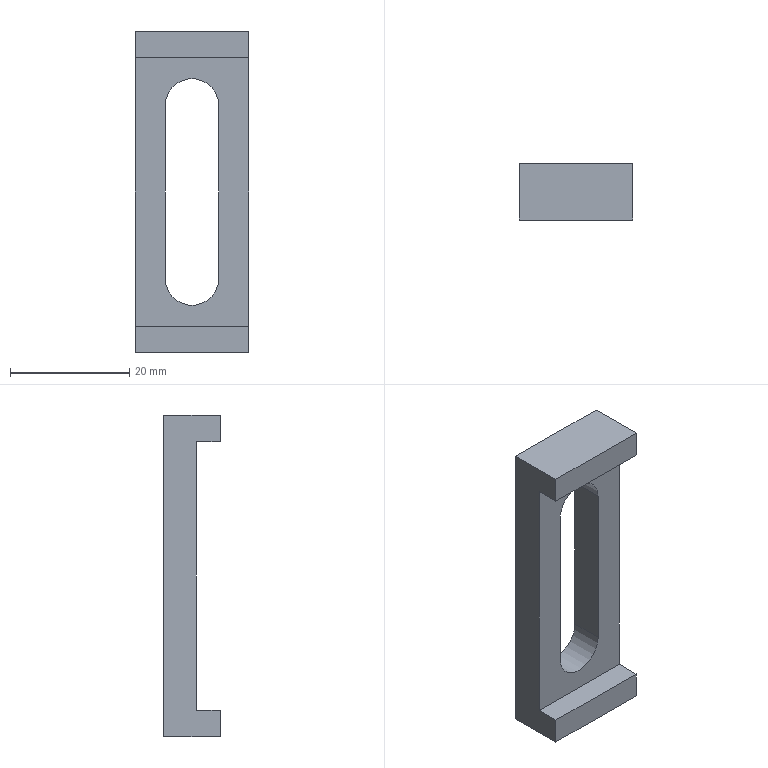Component | NX | SIDE_SUPPORT_FRAME | 1 solid | 14 faces | box 19 x 9.5 x 54 mm | volume 4542 mm3 | plane 12 | cylinder 2 | commonest cylinder face diameters 9 x2
STEP:
#1=CARTESIAN_POINT('',(0.,0.,0.));
#2=DIRECTION('',(0.,0.,1.));
#3=DIRECTION('',(1.,0.,0.));
#4=AXIS2_PLACEMENT_3D('',#1,#2,#3);
#5=CARTESIAN_POINT('',(-95.,46.,111.498));
#6=VERTEX_POINT('',#5);
#7=CARTESIAN_POINT('',(-95.,46.,115.998));
#8=VERTEX_POINT('',#7);
#9=CARTESIAN_POINT('',(-95.,46.,111.498));
#10=DIRECTION('',(0.,0.,1.));
#11=VECTOR('',#10,1.);
#12=LINE('',#9,#11);
#13=CARTESIAN_POINT('',(-104.5,46.,138.498));
#14=DIRECTION('',(0.,-1.,0.));
#15=DIRECTION('',(0.,0.,-1.));
#16=AXIS2_PLACEMENT_3D('',#13,#14,#15);
#17=PLANE('',#16);
#18=CARTESIAN_POINT('',(27.,9.5));
#19=DIRECTION('',(-1.,0.));
#20=VECTOR('',#19,1.);
#21=LINE('',#18,#20);
#22=(GEOMETRIC_REPRESENTATION_CONTEXT(2)PARAMETRIC_REPRESENTATION_CONTEXT()REPRESENTATION_CONTEXT('',''));
#23=DEFINITIONAL_REPRESENTATION('',(#21),#22);
#24=PCURVE('',#17,#23);
#25=CARTESIAN_POINT('',(-95.,46.,111.498));
#26=DIRECTION('',(-1.,0.,0.));
#27=DIRECTION('',(0.,0.,-1.));
#28=AXIS2_PLACEMENT_3D('',#25,#26,#27);
#29=PLANE('',#28);
#30=CARTESIAN_POINT('',(0.,0.));
#31=DIRECTION('',(-1.,0.));
#32=VECTOR('',#31,1.);
#33=LINE('',#30,#32);
#34=(GEOMETRIC_REPRESENTATION_CONTEXT(2)PARAMETRIC_REPRESENTATION_CONTEXT()REPRESENTATION_CONTEXT('',''));
#35=DEFINITIONAL_REPRESENTATION('',(#33),#34);
#36=PCURVE('',#29,#35);
#37=SURFACE_CURVE('',#12,(#24,#36),.PCURVE_S1.);
#38=EDGE_CURVE('',#6,#8,#37,.T.);
#39=ORIENTED_EDGE('',*,*,#38,.T.);
#40=CARTESIAN_POINT('',(-114.,46.,115.998));
#41=VERTEX_POINT('',#40);
#42=CARTESIAN_POINT('',(-94.,46.,115.998));
#43=DIRECTION('',(-1.,0.,0.));
#44=VECTOR('',#43,1.);
#45=LINE('',#42,#44);
#46=CARTESIAN_POINT('',(22.5,10.5));
#47=DIRECTION('',(0.,-1.));
#48=VECTOR('',#47,1.);
#49=LINE('',#46,#48);
#50=(GEOMETRIC_REPRESENTATION_CONTEXT(2)PARAMETRIC_REPRESENTATION_CONTEXT()REPRESENTATION_CONTEXT('',''));
#51=DEFINITIONAL_REPRESENTATION('',(#49),#50);
#52=PCURVE('',#17,#51);
#53=CARTESIAN_POINT('',(-94.,50.,115.998));
#54=DIRECTION('',(0.,0.,-1.));
#55=DIRECTION('',(0.,1.,0.));
#56=AXIS2_PLACEMENT_3D('',#53,#54,#55);
#57=PLANE('',#56);
#58=CARTESIAN_POINT('',(-4.,0.));
#59=DIRECTION('',(0.,-1.));
#60=VECTOR('',#59,1.);
#61=LINE('',#58,#60);
#62=(GEOMETRIC_REPRESENTATION_CONTEXT(2)PARAMETRIC_REPRESENTATION_CONTEXT()REPRESENTATION_CONTEXT('',''));
#63=DEFINITIONAL_REPRESENTATION('',(#61),#62);
#64=PCURVE('',#57,#63);
#65=SURFACE_CURVE('',#45,(#52,#64),.PCURVE_S1.);
#66=EDGE_CURVE('',#8,#41,#65,.T.);
#67=ORIENTED_EDGE('',*,*,#66,.T.);
#68=CARTESIAN_POINT('',(-114.,46.,111.498));
#69=VERTEX_POINT('',#68);
#70=CARTESIAN_POINT('',(-114.,46.,165.498));
#71=DIRECTION('',(0.,0.,-1.));
#72=VECTOR('',#71,1.);
#73=LINE('',#70,#72);
#74=CARTESIAN_POINT('',(-27.,-9.5));
#75=DIRECTION('',(1.,0.));
#76=VECTOR('',#75,1.);
#77=LINE('',#74,#76);
#78=(GEOMETRIC_REPRESENTATION_CONTEXT(2)PARAMETRIC_REPRESENTATION_CONTEXT()REPRESENTATION_CONTEXT('',''));
#79=DEFINITIONAL_REPRESENTATION('',(#77),#78);
#80=PCURVE('',#17,#79);
#81=CARTESIAN_POINT('',(-114.,46.,165.498));
#82=DIRECTION('',(1.,0.,0.));
#83=DIRECTION('',(0.,0.,1.));
#84=AXIS2_PLACEMENT_3D('',#81,#82,#83);
#85=PLANE('',#84);
#86=CARTESIAN_POINT('',(0.,0.));
#87=DIRECTION('',(-1.,0.));
#88=VECTOR('',#87,1.);
#89=LINE('',#86,#88);
#90=(GEOMETRIC_REPRESENTATION_CONTEXT(2)PARAMETRIC_REPRESENTATION_CONTEXT()REPRESENTATION_CONTEXT('',''));
#91=DEFINITIONAL_REPRESENTATION('',(#89),#90);
#92=PCURVE('',#85,#91);
#93=SURFACE_CURVE('',#73,(#80,#92),.PCURVE_S1.);
#94=EDGE_CURVE('',#41,#69,#93,.T.);
#95=ORIENTED_EDGE('',*,*,#94,.T.);
#96=CARTESIAN_POINT('',(-114.,46.,111.498));
#97=DIRECTION('',(1.,0.,0.));
#98=VECTOR('',#97,1.);
#99=LINE('',#96,#98);
#100=CARTESIAN_POINT('',(27.,-9.5));
#101=DIRECTION('',(0.,1.));
#102=VECTOR('',#101,1.);
#103=LINE('',#100,#102);
#104=(GEOMETRIC_REPRESENTATION_CONTEXT(2)PARAMETRIC_REPRESENTATION_CONTEXT()REPRESENTATION_CONTEXT('',''));
#105=DEFINITIONAL_REPRESENTATION('',(#103),#104);
#106=PCURVE('',#17,#105);
#107=CARTESIAN_POINT('',(-114.,46.,111.498));
#108=DIRECTION('',(0.,0.,1.));
#109=DIRECTION('',(0.,-1.,0.));
#110=AXIS2_PLACEMENT_3D('',#107,#108,#109);
#111=PLANE('',#110);
#112=CARTESIAN_POINT('',(0.,0.));
#113=DIRECTION('',(0.,1.));
#114=VECTOR('',#113,1.);
#115=LINE('',#112,#114);
#116=(GEOMETRIC_REPRESENTATION_CONTEXT(2)PARAMETRIC_REPRESENTATION_CONTEXT()REPRESENTATION_CONTEXT('',''));
#117=DEFINITIONAL_REPRESENTATION('',(#115),#116);
#118=PCURVE('',#111,#117);
#119=SURFACE_CURVE('',#99,(#106,#118),.PCURVE_S1.);
#120=EDGE_CURVE('',#69,#6,#119,.T.);
#121=ORIENTED_EDGE('',*,*,#120,.T.);
#122=EDGE_LOOP('',(#39,#67,#95,#121));
#123=FACE_BOUND('',#122,.T.);
#124=ADVANCED_FACE('',(#123),#17,.T.);
#125=CARTESIAN_POINT('',(-114.,50.,115.998));
#126=VERTEX_POINT('',#125);
#127=CARTESIAN_POINT('',(-114.,50.,115.998));
#128=DIRECTION('',(0.,-1.,0.));
#129=VECTOR('',#128,1.);
#130=LINE('',#127,#129);
#131=CARTESIAN_POINT('',(-49.5,-4.));
#132=DIRECTION('',(0.,1.));
#133=VECTOR('',#132,1.);
#134=LINE('',#131,#133);
#135=(GEOMETRIC_REPRESENTATION_CONTEXT(2)PARAMETRIC_REPRESENTATION_CONTEXT()REPRESENTATION_CONTEXT('',''));
#136=DEFINITIONAL_REPRESENTATION('',(#134),#135);
#137=PCURVE('',#85,#136);
#138=CARTESIAN_POINT('',(0.,-20.));
#139=DIRECTION('',(-1.,0.));
#140=VECTOR('',#139,1.);
#141=LINE('',#138,#140);
#142=(GEOMETRIC_REPRESENTATION_CONTEXT(2)PARAMETRIC_REPRESENTATION_CONTEXT()REPRESENTATION_CONTEXT('',''));
#143=DEFINITIONAL_REPRESENTATION('',(#141),#142);
#144=PCURVE('',#57,#143);
#145=SURFACE_CURVE('',#130,(#137,#144),.PCURVE_S1.);
#146=EDGE_CURVE('',#126,#41,#145,.T.);
#147=ORIENTED_EDGE('',*,*,#146,.F.);
#148=CARTESIAN_POINT('',(-114.,50.,160.998));
#149=VERTEX_POINT('',#148);
#150=CARTESIAN_POINT('',(-114.,50.,160.998));
#151=DIRECTION('',(0.,-0.,-1.));
#152=VECTOR('',#151,1.);
#153=LINE('',#150,#152);
#154=CARTESIAN_POINT('',(-4.5,-4.));
#155=DIRECTION('',(-1.,0.));
#156=VECTOR('',#155,1.);
#157=LINE('',#154,#156);
#158=(GEOMETRIC_REPRESENTATION_CONTEXT(2)PARAMETRIC_REPRESENTATION_CONTEXT()REPRESENTATION_CONTEXT('',''));
#159=DEFINITIONAL_REPRESENTATION('',(#157),#158);
#160=PCURVE('',#85,#159);
#161=CARTESIAN_POINT('',(-94.,50.,160.998));
#162=DIRECTION('',(0.,1.,-0.));
#163=DIRECTION('',(0.,0.,1.));
#164=AXIS2_PLACEMENT_3D('',#161,#162,#163);
#165=PLANE('',#164);
#166=CARTESIAN_POINT('',(0.,-20.));
#167=DIRECTION('',(-1.,0.));
#168=VECTOR('',#167,1.);
#169=LINE('',#166,#168);
#170=(GEOMETRIC_REPRESENTATION_CONTEXT(2)PARAMETRIC_REPRESENTATION_CONTEXT()REPRESENTATION_CONTEXT('',''));
#171=DEFINITIONAL_REPRESENTATION('',(#169),#170);
#172=PCURVE('',#165,#171);
#173=SURFACE_CURVE('',#153,(#160,#172),.PCURVE_S1.);
#174=EDGE_CURVE('',#149,#126,#173,.T.);
#175=ORIENTED_EDGE('',*,*,#174,.F.);
#176=CARTESIAN_POINT('',(-114.,46.,160.998));
#177=VERTEX_POINT('',#176);
#178=CARTESIAN_POINT('',(-114.,46.,160.998));
#179=DIRECTION('',(0.,1.,0.));
#180=VECTOR('',#179,1.);
#181=LINE('',#178,#180);
#182=CARTESIAN_POINT('',(-4.5,0.));
#183=DIRECTION('',(0.,-1.));
#184=VECTOR('',#183,1.);
#185=LINE('',#182,#184);
#186=(GEOMETRIC_REPRESENTATION_CONTEXT(2)PARAMETRIC_REPRESENTATION_CONTEXT()REPRESENTATION_CONTEXT('',''));
#187=DEFINITIONAL_REPRESENTATION('',(#185),#186);
#188=PCURVE('',#85,#187);
#189=CARTESIAN_POINT('',(-94.,46.,160.998));
#190=DIRECTION('',(0.,0.,1.));
#191=DIRECTION('',(0.,-1.,0.));
#192=AXIS2_PLACEMENT_3D('',#189,#190,#191);
#193=PLANE('',#192);
#194=CARTESIAN_POINT('',(0.,-20.));
#195=DIRECTION('',(-1.,0.));
#196=VECTOR('',#195,1.);
#197=LINE('',#194,#196);
#198=(GEOMETRIC_REPRESENTATION_CONTEXT(2)PARAMETRIC_REPRESENTATION_CONTEXT()REPRESENTATION_CONTEXT('',''));
#199=DEFINITIONAL_REPRESENTATION('',(#197),#198);
#200=PCURVE('',#193,#199);
#201=SURFACE_CURVE('',#181,(#188,#200),.PCURVE_S1.);
#202=EDGE_CURVE('',#177,#149,#201,.T.);
#203=ORIENTED_EDGE('',*,*,#202,.F.);
#204=CARTESIAN_POINT('',(-114.,46.,165.498));
#205=VERTEX_POINT('',#204);
#206=CARTESIAN_POINT('',(-114.,46.,165.498));
#207=DIRECTION('',(0.,0.,-1.));
#208=VECTOR('',#207,1.);
#209=LINE('',#206,#208);
#210=CARTESIAN_POINT('',(0.,0.));
#211=DIRECTION('',(-1.,0.));
#212=VECTOR('',#211,1.);
#213=LINE('',#210,#212);
#214=(GEOMETRIC_REPRESENTATION_CONTEXT(2)PARAMETRIC_REPRESENTATION_CONTEXT()REPRESENTATION_CONTEXT('',''));
#215=DEFINITIONAL_REPRESENTATION('',(#213),#214);
#216=PCURVE('',#85,#215);
#217=CARTESIAN_POINT('',(-104.5,46.,138.498));
#218=DIRECTION('',(0.,-1.,0.));
#219=DIRECTION('',(0.,0.,-1.));
#220=AXIS2_PLACEMENT_3D('',#217,#218,#219);
#221=PLANE('',#220);
#222=CARTESIAN_POINT('',(-27.,-9.5));
#223=DIRECTION('',(1.,0.));
#224=VECTOR('',#223,1.);
#225=LINE('',#222,#224);
#226=(GEOMETRIC_REPRESENTATION_CONTEXT(2)PARAMETRIC_REPRESENTATION_CONTEXT()REPRESENTATION_CONTEXT('',''));
#227=DEFINITIONAL_REPRESENTATION('',(#225),#226);
#228=PCURVE('',#221,#227);
#229=SURFACE_CURVE('',#209,(#216,#228),.PCURVE_S1.);
#230=EDGE_CURVE('',#205,#177,#229,.T.);
#231=ORIENTED_EDGE('',*,*,#230,.F.);
#232=CARTESIAN_POINT('',(-114.,55.5,165.498));
#233=VERTEX_POINT('',#232);
#234=CARTESIAN_POINT('',(-114.,46.,165.498));
#235=DIRECTION('',(0.,1.,0.));
#236=VECTOR('',#235,1.);
#237=LINE('',#234,#236);
#238=CARTESIAN_POINT('',(0.,0.));
#239=DIRECTION('',(0.,-1.));
#240=VECTOR('',#239,1.);
#241=LINE('',#238,#240);
#242=(GEOMETRIC_REPRESENTATION_CONTEXT(2)PARAMETRIC_REPRESENTATION_CONTEXT()REPRESENTATION_CONTEXT('',''));
#243=DEFINITIONAL_REPRESENTATION('',(#241),#242);
#244=PCURVE('',#85,#243);
#245=CARTESIAN_POINT('',(-95.,46.,165.498));
#246=DIRECTION('',(0.,0.,-1.));
#247=DIRECTION('',(0.,1.,0.));
#248=AXIS2_PLACEMENT_3D('',#245,#246,#247);
#249=PLANE('',#248);
#250=CARTESIAN_POINT('',(0.,-19.));
#251=DIRECTION('',(1.,0.));
#252=VECTOR('',#251,1.);
#253=LINE('',#250,#252);
#254=(GEOMETRIC_REPRESENTATION_CONTEXT(2)PARAMETRIC_REPRESENTATION_CONTEXT()REPRESENTATION_CONTEXT('',''));
#255=DEFINITIONAL_REPRESENTATION('',(#253),#254);
#256=PCURVE('',#249,#255);
#257=SURFACE_CURVE('',#237,(#244,#256),.PCURVE_S1.);
#258=EDGE_CURVE('',#205,#233,#257,.T.);
#259=ORIENTED_EDGE('',*,*,#258,.T.);
#260=CARTESIAN_POINT('',(-114.,55.5,111.498));
#261=VERTEX_POINT('',#260);
#262=CARTESIAN_POINT('',(-114.,55.5,165.498));
#263=DIRECTION('',(0.,0.,-1.));
#264=VECTOR('',#263,1.);
#265=LINE('',#262,#264);
#266=CARTESIAN_POINT('',(0.,-9.5));
#267=DIRECTION('',(-1.,0.));
#268=VECTOR('',#267,1.);
#269=LINE('',#266,#268);
#270=(GEOMETRIC_REPRESENTATION_CONTEXT(2)PARAMETRIC_REPRESENTATION_CONTEXT()REPRESENTATION_CONTEXT('',''));
#271=DEFINITIONAL_REPRESENTATION('',(#269),#270);
#272=PCURVE('',#85,#271);
#273=CARTESIAN_POINT('',(-104.5,55.5,138.498));
#274=DIRECTION('',(0.,-1.,0.));
#275=DIRECTION('',(0.,0.,-1.));
#276=AXIS2_PLACEMENT_3D('',#273,#274,#275);
#277=PLANE('',#276);
#278=CARTESIAN_POINT('',(-27.,-9.5));
#279=DIRECTION('',(1.,0.));
#280=VECTOR('',#279,1.);
#281=LINE('',#278,#280);
#282=(GEOMETRIC_REPRESENTATION_CONTEXT(2)PARAMETRIC_REPRESENTATION_CONTEXT()REPRESENTATION_CONTEXT('',''));
#283=DEFINITIONAL_REPRESENTATION('',(#281),#282);
#284=PCURVE('',#277,#283);
#285=SURFACE_CURVE('',#265,(#272,#284),.PCURVE_S1.);
#286=EDGE_CURVE('',#233,#261,#285,.T.);
#287=ORIENTED_EDGE('',*,*,#286,.T.);
#288=CARTESIAN_POINT('',(-114.,46.,111.498));
#289=DIRECTION('',(0.,1.,0.));
#290=VECTOR('',#289,1.);
#291=LINE('',#288,#290);
#292=CARTESIAN_POINT('',(-54.,0.));
#293=DIRECTION('',(0.,-1.));
#294=VECTOR('',#293,1.);
#295=LINE('',#292,#294);
#296=(GEOMETRIC_REPRESENTATION_CONTEXT(2)PARAMETRIC_REPRESENTATION_CONTEXT()REPRESENTATION_CONTEXT('',''));
#297=DEFINITIONAL_REPRESENTATION('',(#295),#296);
#298=PCURVE('',#85,#297);
#299=CARTESIAN_POINT('',(0.,0.));
#300=DIRECTION('',(-1.,0.));
#301=VECTOR('',#300,1.);
#302=LINE('',#299,#301);
#303=(GEOMETRIC_REPRESENTATION_CONTEXT(2)PARAMETRIC_REPRESENTATION_CONTEXT()REPRESENTATION_CONTEXT('',''));
#304=DEFINITIONAL_REPRESENTATION('',(#302),#303);
#305=PCURVE('',#111,#304);
#306=SURFACE_CURVE('',#291,(#298,#305),.PCURVE_S1.);
#307=EDGE_CURVE('',#69,#261,#306,.T.);
#308=ORIENTED_EDGE('',*,*,#307,.F.);
#309=ORIENTED_EDGE('',*,*,#94,.F.);
#310=EDGE_LOOP('',(#147,#175,#203,#231,#259,#287,#308,#309));
#311=FACE_BOUND('',#310,.T.);
#312=ADVANCED_FACE('',(#311),#85,.F.);
#313=CARTESIAN_POINT('',(-95.,55.5,111.498));
#314=VERTEX_POINT('',#313);
#315=CARTESIAN_POINT('',(-114.,55.5,111.498));
#316=DIRECTION('',(1.,0.,0.));
#317=VECTOR('',#316,1.);
#318=LINE('',#315,#317);
#319=CARTESIAN_POINT('',(-9.5,0.));
#320=DIRECTION('',(0.,1.));
#321=VECTOR('',#320,1.);
#322=LINE('',#319,#321);
#323=(GEOMETRIC_REPRESENTATION_CONTEXT(2)PARAMETRIC_REPRESENTATION_CONTEXT()REPRESENTATION_CONTEXT('',''));
#324=DEFINITIONAL_REPRESENTATION('',(#322),#323);
#325=PCURVE('',#111,#324);
#326=CARTESIAN_POINT('',(27.,-9.5));
#327=DIRECTION('',(0.,1.));
#328=VECTOR('',#327,1.);
#329=LINE('',#326,#328);
#330=(GEOMETRIC_REPRESENTATION_CONTEXT(2)PARAMETRIC_REPRESENTATION_CONTEXT()REPRESENTATION_CONTEXT('',''));
#331=DEFINITIONAL_REPRESENTATION('',(#329),#330);
#332=PCURVE('',#277,#331);
#333=SURFACE_CURVE('',#318,(#325,#332),.PCURVE_S1.);
#334=EDGE_CURVE('',#261,#314,#333,.T.);
#335=ORIENTED_EDGE('',*,*,#334,.T.);
#336=CARTESIAN_POINT('',(-95.,46.,111.498));
#337=DIRECTION('',(0.,1.,0.));
#338=VECTOR('',#337,1.);
#339=LINE('',#336,#338);
#340=CARTESIAN_POINT('',(0.,19.));
#341=DIRECTION('',(-1.,0.));
#342=VECTOR('',#341,1.);
#343=LINE('',#340,#342);
#344=(GEOMETRIC_REPRESENTATION_CONTEXT(2)PARAMETRIC_REPRESENTATION_CONTEXT()REPRESENTATION_CONTEXT('',''));
#345=DEFINITIONAL_REPRESENTATION('',(#343),#344);
#346=PCURVE('',#111,#345);
#347=CARTESIAN_POINT('',(0.,0.));
#348=DIRECTION('',(0.,-1.));
#349=VECTOR('',#348,1.);
#350=LINE('',#347,#349);
#351=(GEOMETRIC_REPRESENTATION_CONTEXT(2)PARAMETRIC_REPRESENTATION_CONTEXT()REPRESENTATION_CONTEXT('',''));
#352=DEFINITIONAL_REPRESENTATION('',(#350),#351);
#353=PCURVE('',#29,#352);
#354=SURFACE_CURVE('',#339,(#346,#353),.PCURVE_S1.);
#355=EDGE_CURVE('',#6,#314,#354,.T.);
#356=ORIENTED_EDGE('',*,*,#355,.F.);
#357=ORIENTED_EDGE('',*,*,#120,.F.);
#358=ORIENTED_EDGE('',*,*,#307,.T.);
#359=EDGE_LOOP('',(#335,#356,#357,#358));
#360=FACE_BOUND('',#359,.T.);
#361=ADVANCED_FACE('',(#360),#111,.F.);
#362=CARTESIAN_POINT('',(-95.,50.,160.998));
#363=VERTEX_POINT('',#362);
#364=CARTESIAN_POINT('',(-95.,50.,115.998));
#365=VERTEX_POINT('',#364);
#366=CARTESIAN_POINT('',(-95.,50.,111.498));
#367=DIRECTION('',(0.,-0.,-1.));
#368=VECTOR('',#367,1.);
#369=LINE('',#366,#368);
#370=CARTESIAN_POINT('',(0.,-4.));
#371=DIRECTION('',(1.,0.));
#372=VECTOR('',#371,1.);
#373=LINE('',#370,#372);
#374=(GEOMETRIC_REPRESENTATION_CONTEXT(2)PARAMETRIC_REPRESENTATION_CONTEXT()REPRESENTATION_CONTEXT('',''));
#375=DEFINITIONAL_REPRESENTATION('',(#373),#374);
#376=PCURVE('',#29,#375);
#377=CARTESIAN_POINT('',(-49.5,-1.));
#378=DIRECTION('',(-1.,0.));
#379=VECTOR('',#378,1.);
#380=LINE('',#377,#379);
#381=(GEOMETRIC_REPRESENTATION_CONTEXT(2)PARAMETRIC_REPRESENTATION_CONTEXT()REPRESENTATION_CONTEXT('',''));
#382=DEFINITIONAL_REPRESENTATION('',(#380),#381);
#383=PCURVE('',#165,#382);
#384=SURFACE_CURVE('',#369,(#376,#383),.PCURVE_S1.);
#385=EDGE_CURVE('',#363,#365,#384,.T.);
#386=ORIENTED_EDGE('',*,*,#385,.T.);
#387=CARTESIAN_POINT('',(-95.,46.,115.998));
#388=DIRECTION('',(0.,-1.,0.));
#389=VECTOR('',#388,1.);
#390=LINE('',#387,#389);
#391=CARTESIAN_POINT('',(-4.5,0.));
#392=DIRECTION('',(0.,1.));
#393=VECTOR('',#392,1.);
#394=LINE('',#391,#393);
#395=(GEOMETRIC_REPRESENTATION_CONTEXT(2)PARAMETRIC_REPRESENTATION_CONTEXT()REPRESENTATION_CONTEXT('',''));
#396=DEFINITIONAL_REPRESENTATION('',(#394),#395);
#397=PCURVE('',#29,#396);
#398=CARTESIAN_POINT('',(-4.,-1.));
#399=DIRECTION('',(-1.,0.));
#400=VECTOR('',#399,1.);
#401=LINE('',#398,#400);
#402=(GEOMETRIC_REPRESENTATION_CONTEXT(2)PARAMETRIC_REPRESENTATION_CONTEXT()REPRESENTATION_CONTEXT('',''));
#403=DEFINITIONAL_REPRESENTATION('',(#401),#402);
#404=PCURVE('',#57,#403);
#405=SURFACE_CURVE('',#390,(#397,#404),.PCURVE_S1.);
#406=EDGE_CURVE('',#365,#8,#405,.T.);
#407=ORIENTED_EDGE('',*,*,#406,.T.);
#408=ORIENTED_EDGE('',*,*,#38,.F.);
#409=ORIENTED_EDGE('',*,*,#355,.T.);
#410=CARTESIAN_POINT('',(-95.,55.5,165.498));
#411=VERTEX_POINT('',#410);
#412=CARTESIAN_POINT('',(-95.,55.5,111.498));
#413=DIRECTION('',(0.,0.,1.));
#414=VECTOR('',#413,1.);
#415=LINE('',#412,#414);
#416=CARTESIAN_POINT('',(0.,-9.5));
#417=DIRECTION('',(-1.,0.));
#418=VECTOR('',#417,1.);
#419=LINE('',#416,#418);
#420=(GEOMETRIC_REPRESENTATION_CONTEXT(2)PARAMETRIC_REPRESENTATION_CONTEXT()REPRESENTATION_CONTEXT('',''));
#421=DEFINITIONAL_REPRESENTATION('',(#419),#420);
#422=PCURVE('',#29,#421);
#423=CARTESIAN_POINT('',(27.,9.5));
#424=DIRECTION('',(-1.,0.));
#425=VECTOR('',#424,1.);
#426=LINE('',#423,#425);
#427=(GEOMETRIC_REPRESENTATION_CONTEXT(2)PARAMETRIC_REPRESENTATION_CONTEXT()REPRESENTATION_CONTEXT('',''));
#428=DEFINITIONAL_REPRESENTATION('',(#426),#427);
#429=PCURVE('',#277,#428);
#430=SURFACE_CURVE('',#415,(#422,#429),.PCURVE_S1.);
#431=EDGE_CURVE('',#314,#411,#430,.T.);
#432=ORIENTED_EDGE('',*,*,#431,.T.);
#433=CARTESIAN_POINT('',(-95.,46.,165.498));
#434=VERTEX_POINT('',#433);
#435=CARTESIAN_POINT('',(-95.,46.,165.498));
#436=DIRECTION('',(0.,1.,0.));
#437=VECTOR('',#436,1.);
#438=LINE('',#435,#437);
#439=CARTESIAN_POINT('',(-54.,0.));
#440=DIRECTION('',(0.,-1.));
#441=VECTOR('',#440,1.);
#442=LINE('',#439,#441);
#443=(GEOMETRIC_REPRESENTATION_CONTEXT(2)PARAMETRIC_REPRESENTATION_CONTEXT()REPRESENTATION_CONTEXT('',''));
#444=DEFINITIONAL_REPRESENTATION('',(#442),#443);
#445=PCURVE('',#29,#444);
#446=CARTESIAN_POINT('',(0.,0.));
#447=DIRECTION('',(1.,0.));
#448=VECTOR('',#447,1.);
#449=LINE('',#446,#448);
#450=(GEOMETRIC_REPRESENTATION_CONTEXT(2)PARAMETRIC_REPRESENTATION_CONTEXT()REPRESENTATION_CONTEXT('',''));
#451=DEFINITIONAL_REPRESENTATION('',(#449),#450);
#452=PCURVE('',#249,#451);
#453=SURFACE_CURVE('',#438,(#445,#452),.PCURVE_S1.);
#454=EDGE_CURVE('',#434,#411,#453,.T.);
#455=ORIENTED_EDGE('',*,*,#454,.F.);
#456=CARTESIAN_POINT('',(-95.,46.,160.998));
#457=VERTEX_POINT('',#456);
#458=CARTESIAN_POINT('',(-95.,46.,111.498));
#459=DIRECTION('',(0.,0.,1.));
#460=VECTOR('',#459,1.);
#461=LINE('',#458,#460);
#462=CARTESIAN_POINT('',(0.,0.));
#463=DIRECTION('',(-1.,0.));
#464=VECTOR('',#463,1.);
#465=LINE('',#462,#464);
#466=(GEOMETRIC_REPRESENTATION_CONTEXT(2)PARAMETRIC_REPRESENTATION_CONTEXT()REPRESENTATION_CONTEXT('',''));
#467=DEFINITIONAL_REPRESENTATION('',(#465),#466);
#468=PCURVE('',#29,#467);
#469=CARTESIAN_POINT('',(27.,9.5));
#470=DIRECTION('',(-1.,0.));
#471=VECTOR('',#470,1.);
#472=LINE('',#469,#471);
#473=(GEOMETRIC_REPRESENTATION_CONTEXT(2)PARAMETRIC_REPRESENTATION_CONTEXT()REPRESENTATION_CONTEXT('',''));
#474=DEFINITIONAL_REPRESENTATION('',(#472),#473);
#475=PCURVE('',#221,#474);
#476=SURFACE_CURVE('',#461,(#468,#475),.PCURVE_S1.);
#477=EDGE_CURVE('',#457,#434,#476,.T.);
#478=ORIENTED_EDGE('',*,*,#477,.F.);
#479=CARTESIAN_POINT('',(-95.,46.,160.998));
#480=DIRECTION('',(0.,1.,0.));
#481=VECTOR('',#480,1.);
#482=LINE('',#479,#481);
#483=CARTESIAN_POINT('',(-49.5,0.));
#484=DIRECTION('',(0.,-1.));
#485=VECTOR('',#484,1.);
#486=LINE('',#483,#485);
#487=(GEOMETRIC_REPRESENTATION_CONTEXT(2)PARAMETRIC_REPRESENTATION_CONTEXT()REPRESENTATION_CONTEXT('',''));
#488=DEFINITIONAL_REPRESENTATION('',(#486),#487);
#489=PCURVE('',#29,#488);
#490=CARTESIAN_POINT('',(0.,-1.));
#491=DIRECTION('',(-1.,0.));
#492=VECTOR('',#491,1.);
#493=LINE('',#490,#492);
#494=(GEOMETRIC_REPRESENTATION_CONTEXT(2)PARAMETRIC_REPRESENTATION_CONTEXT()REPRESENTATION_CONTEXT('',''));
#495=DEFINITIONAL_REPRESENTATION('',(#493),#494);
#496=PCURVE('',#193,#495);
#497=SURFACE_CURVE('',#482,(#489,#496),.PCURVE_S1.);
#498=EDGE_CURVE('',#457,#363,#497,.T.);
#499=ORIENTED_EDGE('',*,*,#498,.T.);
#500=EDGE_LOOP('',(#386,#407,#408,#409,#432,#455,#478,#499));
#501=FACE_BOUND('',#500,.T.);
#502=ADVANCED_FACE('',(#501),#29,.F.);
#503=CARTESIAN_POINT('',(-95.,55.5,165.498));
#504=DIRECTION('',(-1.,0.,0.));
#505=VECTOR('',#504,1.);
#506=LINE('',#503,#505);
#507=CARTESIAN_POINT('',(9.5,0.));
#508=DIRECTION('',(0.,-1.));
#509=VECTOR('',#508,1.);
#510=LINE('',#507,#509);
#511=(GEOMETRIC_REPRESENTATION_CONTEXT(2)PARAMETRIC_REPRESENTATION_CONTEXT()REPRESENTATION_CONTEXT('',''));
#512=DEFINITIONAL_REPRESENTATION('',(#510),#511);
#513=PCURVE('',#249,#512);
#514=CARTESIAN_POINT('',(-27.,9.5));
#515=DIRECTION('',(0.,-1.));
#516=VECTOR('',#515,1.);
#517=LINE('',#514,#516);
#518=(GEOMETRIC_REPRESENTATION_CONTEXT(2)PARAMETRIC_REPRESENTATION_CONTEXT()REPRESENTATION_CONTEXT('',''));
#519=DEFINITIONAL_REPRESENTATION('',(#517),#518);
#520=PCURVE('',#277,#519);
#521=SURFACE_CURVE('',#506,(#513,#520),.PCURVE_S1.);
#522=EDGE_CURVE('',#411,#233,#521,.T.);
#523=ORIENTED_EDGE('',*,*,#522,.T.);
#524=ORIENTED_EDGE('',*,*,#258,.F.);
#525=CARTESIAN_POINT('',(-95.,46.,165.498));
#526=DIRECTION('',(-1.,0.,0.));
#527=VECTOR('',#526,1.);
#528=LINE('',#525,#527);
#529=CARTESIAN_POINT('',(0.,0.));
#530=DIRECTION('',(0.,-1.));
#531=VECTOR('',#530,1.);
#532=LINE('',#529,#531);
#533=(GEOMETRIC_REPRESENTATION_CONTEXT(2)PARAMETRIC_REPRESENTATION_CONTEXT()REPRESENTATION_CONTEXT('',''));
#534=DEFINITIONAL_REPRESENTATION('',(#532),#533);
#535=PCURVE('',#249,#534);
#536=CARTESIAN_POINT('',(-27.,9.5));
#537=DIRECTION('',(0.,-1.));
#538=VECTOR('',#537,1.);
#539=LINE('',#536,#538);
#540=(GEOMETRIC_REPRESENTATION_CONTEXT(2)PARAMETRIC_REPRESENTATION_CONTEXT()REPRESENTATION_CONTEXT('',''));
#541=DEFINITIONAL_REPRESENTATION('',(#539),#540);
#542=PCURVE('',#221,#541);
#543=SURFACE_CURVE('',#528,(#535,#542),.PCURVE_S1.);
#544=EDGE_CURVE('',#434,#205,#543,.T.);
#545=ORIENTED_EDGE('',*,*,#544,.F.);
#546=ORIENTED_EDGE('',*,*,#454,.T.);
#547=EDGE_LOOP('',(#523,#524,#545,#546));
#548=FACE_BOUND('',#547,.T.);
#549=ADVANCED_FACE('',(#548),#249,.F.);
#550=CARTESIAN_POINT('',(-94.,46.,160.998));
#551=DIRECTION('',(-1.,0.,0.));
#552=VECTOR('',#551,1.);
#553=LINE('',#550,#552);
#554=CARTESIAN_POINT('',(-22.5,10.5));
#555=DIRECTION('',(0.,-1.));
#556=VECTOR('',#555,1.);
#557=LINE('',#554,#556);
#558=(GEOMETRIC_REPRESENTATION_CONTEXT(2)PARAMETRIC_REPRESENTATION_CONTEXT()REPRESENTATION_CONTEXT('',''));
#559=DEFINITIONAL_REPRESENTATION('',(#557),#558);
#560=PCURVE('',#221,#559);
#561=CARTESIAN_POINT('',(0.,0.));
#562=DIRECTION('',(0.,-1.));
#563=VECTOR('',#562,1.);
#564=LINE('',#561,#563);
#565=(GEOMETRIC_REPRESENTATION_CONTEXT(2)PARAMETRIC_REPRESENTATION_CONTEXT()REPRESENTATION_CONTEXT('',''));
#566=DEFINITIONAL_REPRESENTATION('',(#564),#565);
#567=PCURVE('',#193,#566);
#568=SURFACE_CURVE('',#553,(#560,#567),.PCURVE_S1.);
#569=EDGE_CURVE('',#457,#177,#568,.T.);
#570=ORIENTED_EDGE('',*,*,#569,.F.);
#571=ORIENTED_EDGE('',*,*,#477,.T.);
#572=ORIENTED_EDGE('',*,*,#544,.T.);
#573=ORIENTED_EDGE('',*,*,#230,.T.);
#574=EDGE_LOOP('',(#570,#571,#572,#573));
#575=FACE_BOUND('',#574,.T.);
#576=ADVANCED_FACE('',(#575),#221,.T.);
#577=CARTESIAN_POINT('',(-100.,55.5,152.998));
#578=VERTEX_POINT('',#577);
#579=CARTESIAN_POINT('',(-109.,55.5,152.998));
#580=VERTEX_POINT('',#579);
#581=CARTESIAN_POINT('',(-104.5,55.5,152.998));
#582=DIRECTION('',(0.,-1.,0.));
#583=DIRECTION('',(0.,0.,-1.));
#584=AXIS2_PLACEMENT_3D('',#581,#582,#583);
#585=CIRCLE('',#584,4.5);
#586=CARTESIAN_POINT('',(-14.5,0.));
#587=DIRECTION('',(1.,0.));
#588=AXIS2_PLACEMENT_2D('',#586,#587);
#589=CIRCLE('',#588,4.5);
#590=(GEOMETRIC_REPRESENTATION_CONTEXT(2)PARAMETRIC_REPRESENTATION_CONTEXT()REPRESENTATION_CONTEXT('',''));
#591=DEFINITIONAL_REPRESENTATION('',(#589),#590);
#592=PCURVE('',#277,#591);
#593=CARTESIAN_POINT('',(-104.5,70.,152.998));
#594=DIRECTION('',(0.,-1.,0.));
#595=DIRECTION('',(0.,-0.,-1.));
#596=AXIS2_PLACEMENT_3D('',#593,#594,#595);
#597=CYLINDRICAL_SURFACE('',#596,4.5);
#598=CARTESIAN_POINT('',(-0.,14.5));
#599=DIRECTION('',(1.,0.));
#600=VECTOR('',#599,1.);
#601=LINE('',#598,#600);
#602=(GEOMETRIC_REPRESENTATION_CONTEXT(2)PARAMETRIC_REPRESENTATION_CONTEXT()REPRESENTATION_CONTEXT('',''));
#603=DEFINITIONAL_REPRESENTATION('',(#601),#602);
#604=PCURVE('',#597,#603);
#605=SURFACE_CURVE('',#585,(#592,#604),.PCURVE_S1.);
#606=EDGE_CURVE('',#578,#580,#605,.T.);
#607=ORIENTED_EDGE('',*,*,#606,.T.);
#608=CARTESIAN_POINT('',(-109.,55.5,123.998));
#609=VERTEX_POINT('',#608);
#610=CARTESIAN_POINT('',(-109.,55.5,138.498));
#611=DIRECTION('',(0.,0.,-1.));
#612=VECTOR('',#611,1.);
#613=LINE('',#610,#612);
#614=CARTESIAN_POINT('',(0.,-4.5));
#615=DIRECTION('',(1.,0.));
#616=VECTOR('',#615,1.);
#617=LINE('',#614,#616);
#618=(GEOMETRIC_REPRESENTATION_CONTEXT(2)PARAMETRIC_REPRESENTATION_CONTEXT()REPRESENTATION_CONTEXT('',''));
#619=DEFINITIONAL_REPRESENTATION('',(#617),#618);
#620=PCURVE('',#277,#619);
#621=CARTESIAN_POINT('',(-109.,70.,152.998));
#622=DIRECTION('',(-1.,0.,0.));
#623=DIRECTION('',(0.,0.,-1.));
#624=AXIS2_PLACEMENT_3D('',#621,#622,#623);
#625=PLANE('',#624);
#626=CARTESIAN_POINT('',(14.5,14.5));
#627=DIRECTION('',(1.,0.));
#628=VECTOR('',#627,1.);
#629=LINE('',#626,#628);
#630=(GEOMETRIC_REPRESENTATION_CONTEXT(2)PARAMETRIC_REPRESENTATION_CONTEXT()REPRESENTATION_CONTEXT('',''));
#631=DEFINITIONAL_REPRESENTATION('',(#629),#630);
#632=PCURVE('',#625,#631);
#633=SURFACE_CURVE('',#613,(#620,#632),.PCURVE_S1.);
#634=EDGE_CURVE('',#580,#609,#633,.T.);
#635=ORIENTED_EDGE('',*,*,#634,.T.);
#636=CARTESIAN_POINT('',(-100.,55.5,123.998));
#637=VERTEX_POINT('',#636);
#638=CARTESIAN_POINT('',(-104.5,55.5,123.998));
#639=DIRECTION('',(0.,-1.,0.));
#640=DIRECTION('',(0.,0.,-1.));
#641=AXIS2_PLACEMENT_3D('',#638,#639,#640);
#642=CIRCLE('',#641,4.5);
#643=CARTESIAN_POINT('',(14.5,0.));
#644=DIRECTION('',(1.,0.));
#645=AXIS2_PLACEMENT_2D('',#643,#644);
#646=CIRCLE('',#645,4.5);
#647=(GEOMETRIC_REPRESENTATION_CONTEXT(2)PARAMETRIC_REPRESENTATION_CONTEXT()REPRESENTATION_CONTEXT('',''));
#648=DEFINITIONAL_REPRESENTATION('',(#646),#647);
#649=PCURVE('',#277,#648);
#650=CARTESIAN_POINT('',(-104.5,70.,123.998));
#651=DIRECTION('',(0.,-1.,0.));
#652=DIRECTION('',(0.,-0.,-1.));
#653=AXIS2_PLACEMENT_3D('',#650,#651,#652);
#654=CYLINDRICAL_SURFACE('',#653,4.5);
#655=CARTESIAN_POINT('',(0.,14.5));
#656=DIRECTION('',(1.,0.));
#657=VECTOR('',#656,1.);
#658=LINE('',#655,#657);
#659=(GEOMETRIC_REPRESENTATION_CONTEXT(2)PARAMETRIC_REPRESENTATION_CONTEXT()REPRESENTATION_CONTEXT('',''));
#660=DEFINITIONAL_REPRESENTATION('',(#658),#659);
#661=PCURVE('',#654,#660);
#662=SURFACE_CURVE('',#642,(#649,#661),.PCURVE_S1.);
#663=EDGE_CURVE('',#609,#637,#662,.T.);
#664=ORIENTED_EDGE('',*,*,#663,.T.);
#665=CARTESIAN_POINT('',(-100.,55.5,138.498));
#666=DIRECTION('',(0.,0.,1.));
#667=VECTOR('',#666,1.);
#668=LINE('',#665,#667);
#669=CARTESIAN_POINT('',(0.,4.5));
#670=DIRECTION('',(-1.,0.));
#671=VECTOR('',#670,1.);
#672=LINE('',#669,#671);
#673=(GEOMETRIC_REPRESENTATION_CONTEXT(2)PARAMETRIC_REPRESENTATION_CONTEXT()REPRESENTATION_CONTEXT('',''));
#674=DEFINITIONAL_REPRESENTATION('',(#672),#673);
#675=PCURVE('',#277,#674);
#676=CARTESIAN_POINT('',(-100.,70.,123.998));
#677=DIRECTION('',(1.,0.,0.));
#678=DIRECTION('',(0.,0.,1.));
#679=AXIS2_PLACEMENT_3D('',#676,#677,#678);
#680=PLANE('',#679);
#681=CARTESIAN_POINT('',(14.5,14.5));
#682=DIRECTION('',(1.,0.));
#683=VECTOR('',#682,1.);
#684=LINE('',#681,#683);
#685=(GEOMETRIC_REPRESENTATION_CONTEXT(2)PARAMETRIC_REPRESENTATION_CONTEXT()REPRESENTATION_CONTEXT('',''));
#686=DEFINITIONAL_REPRESENTATION('',(#684),#685);
#687=PCURVE('',#680,#686);
#688=SURFACE_CURVE('',#668,(#675,#687),.PCURVE_S1.);
#689=EDGE_CURVE('',#637,#578,#688,.T.);
#690=ORIENTED_EDGE('',*,*,#689,.T.);
#691=EDGE_LOOP('',(#607,#635,#664,#690));
#692=FACE_BOUND('',#691,.T.);
#693=ORIENTED_EDGE('',*,*,#286,.F.);
#694=ORIENTED_EDGE('',*,*,#522,.F.);
#695=ORIENTED_EDGE('',*,*,#431,.F.);
#696=ORIENTED_EDGE('',*,*,#334,.F.);
#697=EDGE_LOOP('',(#693,#694,#695,#696));
#698=FACE_BOUND('',#697,.T.);
#699=ADVANCED_FACE('',(#692,#698),#277,.F.);
#700=CARTESIAN_POINT('',(-109.,50.,123.998));
#701=VERTEX_POINT('',#700);
#702=CARTESIAN_POINT('',(-100.,50.,123.998));
#703=VERTEX_POINT('',#702);
#704=CARTESIAN_POINT('',(-104.5,50.,123.998));
#705=DIRECTION('',(0.,-1.,0.));
#706=DIRECTION('',(0.,0.,1.));
#707=AXIS2_PLACEMENT_3D('',#704,#705,#706);
#708=CIRCLE('',#707,4.5);
#709=CARTESIAN_POINT('',(-32.5,-10.5));
#710=CARTESIAN_POINT('',(-32.5,-18.294));
#711=CARTESIAN_POINT('',(-39.25,-14.397));
#712=CARTESIAN_POINT('',(-46.,-10.5));
#713=CARTESIAN_POINT('',(-39.25,-6.603));
#714=CARTESIAN_POINT('',(-32.5,-2.706));
#715=CARTESIAN_POINT('',(-32.5,-10.5));
#716=(BOUNDED_CURVE()B_SPLINE_CURVE(2,(#709,#710,#711,#712,#713,#714,#715),.UNSPECIFIED.,.T.,.F.)B_SPLINE_CURVE_WITH_KNOTS((1,2,2,2,2,1),(-2.094,0.,2.094,4.189,6.283,8.378),.UNSPECIFIED.)CURVE()GEOMETRIC_REPRESENTATION_ITEM()RATIONAL_B_SPLINE_CURVE((1.,0.5,1.,0.5,1.,0.5,1.))REPRESENTATION_ITEM(''));
#717=(GEOMETRIC_REPRESENTATION_CONTEXT(2)PARAMETRIC_REPRESENTATION_CONTEXT()REPRESENTATION_CONTEXT('',''));
#718=DEFINITIONAL_REPRESENTATION('',(#716),#717);
#719=PCURVE('',#165,#718);
#720=CARTESIAN_POINT('',(3.142,20.));
#721=DIRECTION('',(1.,0.));
#722=VECTOR('',#721,1.);
#723=LINE('',#720,#722);
#724=(GEOMETRIC_REPRESENTATION_CONTEXT(2)PARAMETRIC_REPRESENTATION_CONTEXT()REPRESENTATION_CONTEXT('',''));
#725=DEFINITIONAL_REPRESENTATION('',(#723),#724);
#726=PCURVE('',#654,#725);
#727=SURFACE_CURVE('',#708,(#719,#726),.PCURVE_S1.);
#728=EDGE_CURVE('',#701,#703,#727,.T.);
#729=ORIENTED_EDGE('',*,*,#728,.F.);
#730=CARTESIAN_POINT('',(-109.,50.,152.998));
#731=VERTEX_POINT('',#730);
#732=CARTESIAN_POINT('',(-109.,50.,152.998));
#733=DIRECTION('',(0.,-0.,-1.));
#734=VECTOR('',#733,1.);
#735=LINE('',#732,#734);
#736=CARTESIAN_POINT('',(-8.,-15.));
#737=DIRECTION('',(-1.,0.));
#738=VECTOR('',#737,1.);
#739=LINE('',#736,#738);
#740=(GEOMETRIC_REPRESENTATION_CONTEXT(2)PARAMETRIC_REPRESENTATION_CONTEXT()REPRESENTATION_CONTEXT('',''));
#741=DEFINITIONAL_REPRESENTATION('',(#739),#740);
#742=PCURVE('',#165,#741);
#743=CARTESIAN_POINT('',(0.,20.));
#744=DIRECTION('',(1.,0.));
#745=VECTOR('',#744,1.);
#746=LINE('',#743,#745);
#747=(GEOMETRIC_REPRESENTATION_CONTEXT(2)PARAMETRIC_REPRESENTATION_CONTEXT()REPRESENTATION_CONTEXT('',''));
#748=DEFINITIONAL_REPRESENTATION('',(#746),#747);
#749=PCURVE('',#625,#748);
#750=SURFACE_CURVE('',#735,(#742,#749),.PCURVE_S1.);
#751=EDGE_CURVE('',#731,#701,#750,.T.);
#752=ORIENTED_EDGE('',*,*,#751,.F.);
#753=CARTESIAN_POINT('',(-100.,50.,152.998));
#754=VERTEX_POINT('',#753);
#755=CARTESIAN_POINT('',(-104.5,50.,152.998));
#756=DIRECTION('',(0.,-1.,0.));
#757=DIRECTION('',(0.,0.,-1.));
#758=AXIS2_PLACEMENT_3D('',#755,#756,#757);
#759=CIRCLE('',#758,4.5);
#760=CARTESIAN_POINT('',(-12.5,-10.5));
#761=CARTESIAN_POINT('',(-12.5,-2.706));
#762=CARTESIAN_POINT('',(-5.75,-6.603));
#763=CARTESIAN_POINT('',(1.,-10.5));
#764=CARTESIAN_POINT('',(-5.75,-14.397));
#765=CARTESIAN_POINT('',(-12.5,-18.294));
#766=CARTESIAN_POINT('',(-12.5,-10.5));
#767=(BOUNDED_CURVE()B_SPLINE_CURVE(2,(#760,#761,#762,#763,#764,#765,#766),.UNSPECIFIED.,.T.,.F.)B_SPLINE_CURVE_WITH_KNOTS((1,2,2,2,2,1),(-2.094,0.,2.094,4.189,6.283,8.378),.UNSPECIFIED.)CURVE()GEOMETRIC_REPRESENTATION_ITEM()RATIONAL_B_SPLINE_CURVE((1.,0.5,1.,0.5,1.,0.5,1.))REPRESENTATION_ITEM(''));
#768=(GEOMETRIC_REPRESENTATION_CONTEXT(2)PARAMETRIC_REPRESENTATION_CONTEXT()REPRESENTATION_CONTEXT('',''));
#769=DEFINITIONAL_REPRESENTATION('',(#767),#768);
#770=PCURVE('',#165,#769);
#771=CARTESIAN_POINT('',(-0.,20.));
#772=DIRECTION('',(1.,0.));
#773=VECTOR('',#772,1.);
#774=LINE('',#771,#773);
#775=(GEOMETRIC_REPRESENTATION_CONTEXT(2)PARAMETRIC_REPRESENTATION_CONTEXT()REPRESENTATION_CONTEXT('',''));
#776=DEFINITIONAL_REPRESENTATION('',(#774),#775);
#777=PCURVE('',#597,#776);
#778=SURFACE_CURVE('',#759,(#770,#777),.PCURVE_S1.);
#779=EDGE_CURVE('',#754,#731,#778,.T.);
#780=ORIENTED_EDGE('',*,*,#779,.F.);
#781=CARTESIAN_POINT('',(-100.,50.,123.998));
#782=DIRECTION('',(0.,0.,1.));
#783=VECTOR('',#782,1.);
#784=LINE('',#781,#783);
#785=CARTESIAN_POINT('',(-37.,-6.));
#786=DIRECTION('',(1.,0.));
#787=VECTOR('',#786,1.);
#788=LINE('',#785,#787);
#789=(GEOMETRIC_REPRESENTATION_CONTEXT(2)PARAMETRIC_REPRESENTATION_CONTEXT()REPRESENTATION_CONTEXT('',''));
#790=DEFINITIONAL_REPRESENTATION('',(#788),#789);
#791=PCURVE('',#165,#790);
#792=CARTESIAN_POINT('',(0.,20.));
#793=DIRECTION('',(1.,-0.));
#794=VECTOR('',#793,1.);
#795=LINE('',#792,#794);
#796=(GEOMETRIC_REPRESENTATION_CONTEXT(2)PARAMETRIC_REPRESENTATION_CONTEXT()REPRESENTATION_CONTEXT('',''));
#797=DEFINITIONAL_REPRESENTATION('',(#795),#796);
#798=PCURVE('',#680,#797);
#799=SURFACE_CURVE('',#784,(#791,#798),.PCURVE_S1.);
#800=EDGE_CURVE('',#703,#754,#799,.T.);
#801=ORIENTED_EDGE('',*,*,#800,.F.);
#802=EDGE_LOOP('',(#729,#752,#780,#801));
#803=FACE_BOUND('',#802,.T.);
#804=CARTESIAN_POINT('',(-94.,50.,160.998));
#805=DIRECTION('',(1.,0.,0.));
#806=VECTOR('',#805,1.);
#807=LINE('',#804,#806);
#808=CARTESIAN_POINT('',(0.,0.));
#809=DIRECTION('',(0.,1.));
#810=VECTOR('',#809,1.);
#811=LINE('',#808,#810);
#812=(GEOMETRIC_REPRESENTATION_CONTEXT(2)PARAMETRIC_REPRESENTATION_CONTEXT()REPRESENTATION_CONTEXT('',''));
#813=DEFINITIONAL_REPRESENTATION('',(#811),#812);
#814=PCURVE('',#165,#813);
#815=CARTESIAN_POINT('',(-4.,0.));
#816=DIRECTION('',(0.,1.));
#817=VECTOR('',#816,1.);
#818=LINE('',#815,#817);
#819=(GEOMETRIC_REPRESENTATION_CONTEXT(2)PARAMETRIC_REPRESENTATION_CONTEXT()REPRESENTATION_CONTEXT('',''));
#820=DEFINITIONAL_REPRESENTATION('',(#818),#819);
#821=PCURVE('',#193,#820);
#822=SURFACE_CURVE('',#807,(#814,#821),.PCURVE_S1.);
#823=EDGE_CURVE('',#149,#363,#822,.T.);
#824=ORIENTED_EDGE('',*,*,#823,.F.);
#825=ORIENTED_EDGE('',*,*,#174,.T.);
#826=CARTESIAN_POINT('',(-94.,50.,115.998));
#827=DIRECTION('',(1.,0.,0.));
#828=VECTOR('',#827,1.);
#829=LINE('',#826,#828);
#830=CARTESIAN_POINT('',(-45.,0.));
#831=DIRECTION('',(0.,1.));
#832=VECTOR('',#831,1.);
#833=LINE('',#830,#832);
#834=(GEOMETRIC_REPRESENTATION_CONTEXT(2)PARAMETRIC_REPRESENTATION_CONTEXT()REPRESENTATION_CONTEXT('',''));
#835=DEFINITIONAL_REPRESENTATION('',(#833),#834);
#836=PCURVE('',#165,#835);
#837=CARTESIAN_POINT('',(0.,0.));
#838=DIRECTION('',(0.,1.));
#839=VECTOR('',#838,1.);
#840=LINE('',#837,#839);
#841=(GEOMETRIC_REPRESENTATION_CONTEXT(2)PARAMETRIC_REPRESENTATION_CONTEXT()REPRESENTATION_CONTEXT('',''));
#842=DEFINITIONAL_REPRESENTATION('',(#840),#841);
#843=PCURVE('',#57,#842);
#844=SURFACE_CURVE('',#829,(#836,#843),.PCURVE_S1.);
#845=EDGE_CURVE('',#126,#365,#844,.T.);
#846=ORIENTED_EDGE('',*,*,#845,.T.);
#847=ORIENTED_EDGE('',*,*,#385,.F.);
#848=EDGE_LOOP('',(#824,#825,#846,#847));
#849=FACE_BOUND('',#848,.T.);
#850=ADVANCED_FACE('',(#803,#849),#165,.F.);
#851=ORIENTED_EDGE('',*,*,#845,.F.);
#852=ORIENTED_EDGE('',*,*,#146,.T.);
#853=ORIENTED_EDGE('',*,*,#66,.F.);
#854=ORIENTED_EDGE('',*,*,#406,.F.);
#855=EDGE_LOOP('',(#851,#852,#853,#854));
#856=FACE_BOUND('',#855,.T.);
#857=ADVANCED_FACE('',(#856),#57,.F.);
#858=ORIENTED_EDGE('',*,*,#569,.T.);
#859=ORIENTED_EDGE('',*,*,#202,.T.);
#860=ORIENTED_EDGE('',*,*,#823,.T.);
#861=ORIENTED_EDGE('',*,*,#498,.F.);
#862=EDGE_LOOP('',(#858,#859,#860,#861));
#863=FACE_BOUND('',#862,.T.);
#864=ADVANCED_FACE('',(#863),#193,.F.);
#865=CARTESIAN_POINT('',(-109.,70.,152.998));
#866=DIRECTION('',(0.,1.,-0.));
#867=VECTOR('',#866,1.);
#868=LINE('',#865,#867);
#869=CARTESIAN_POINT('',(0.,0.));
#870=DIRECTION('',(0.,-1.));
#871=VECTOR('',#870,1.);
#872=LINE('',#869,#871);
#873=(GEOMETRIC_REPRESENTATION_CONTEXT(2)PARAMETRIC_REPRESENTATION_CONTEXT()REPRESENTATION_CONTEXT('',''));
#874=DEFINITIONAL_REPRESENTATION('',(#872),#873);
#875=PCURVE('',#625,#874);
#876=CARTESIAN_POINT('',(4.712,0.));
#877=DIRECTION('',(0.,-1.));
#878=VECTOR('',#877,1.);
#879=LINE('',#876,#878);
#880=(GEOMETRIC_REPRESENTATION_CONTEXT(2)PARAMETRIC_REPRESENTATION_CONTEXT()REPRESENTATION_CONTEXT('',''));
#881=DEFINITIONAL_REPRESENTATION('',(#879),#880);
#882=PCURVE('',#597,#881);
#883=SURFACE_CURVE('',#868,(#875,#882),.PCURVE_S1.);
#884=EDGE_CURVE('',#731,#580,#883,.T.);
#885=ORIENTED_EDGE('',*,*,#884,.F.);
#886=ORIENTED_EDGE('',*,*,#751,.T.);
#887=CARTESIAN_POINT('',(-109.,70.,123.998));
#888=DIRECTION('',(0.,1.,-0.));
#889=VECTOR('',#888,1.);
#890=LINE('',#887,#889);
#891=CARTESIAN_POINT('',(29.,0.));
#892=DIRECTION('',(0.,-1.));
#893=VECTOR('',#892,1.);
#894=LINE('',#891,#893);
#895=(GEOMETRIC_REPRESENTATION_CONTEXT(2)PARAMETRIC_REPRESENTATION_CONTEXT()REPRESENTATION_CONTEXT('',''));
#896=DEFINITIONAL_REPRESENTATION('',(#894),#895);
#897=PCURVE('',#625,#896);
#898=CARTESIAN_POINT('',(4.712,0.));
#899=DIRECTION('',(0.,-1.));
#900=VECTOR('',#899,1.);
#901=LINE('',#898,#900);
#902=(GEOMETRIC_REPRESENTATION_CONTEXT(2)PARAMETRIC_REPRESENTATION_CONTEXT()REPRESENTATION_CONTEXT('',''));
#903=DEFINITIONAL_REPRESENTATION('',(#901),#902);
#904=PCURVE('',#654,#903);
#905=SURFACE_CURVE('',#890,(#897,#904),.PCURVE_S1.);
#906=EDGE_CURVE('',#701,#609,#905,.T.);
#907=ORIENTED_EDGE('',*,*,#906,.T.);
#908=ORIENTED_EDGE('',*,*,#634,.F.);
#909=EDGE_LOOP('',(#885,#886,#907,#908));
#910=FACE_BOUND('',#909,.T.);
#911=ADVANCED_FACE('',(#910),#625,.F.);
#912=ORIENTED_EDGE('',*,*,#663,.T.);
#913=CARTESIAN_POINT('',(-100.,70.,123.998));
#914=DIRECTION('',(0.,1.,-0.));
#915=VECTOR('',#914,1.);
#916=LINE('',#913,#915);
#917=CARTESIAN_POINT('',(7.854,0.));
#918=DIRECTION('',(0.,-1.));
#919=VECTOR('',#918,1.);
#920=LINE('',#917,#919);
#921=(GEOMETRIC_REPRESENTATION_CONTEXT(2)PARAMETRIC_REPRESENTATION_CONTEXT()REPRESENTATION_CONTEXT('',''));
#922=DEFINITIONAL_REPRESENTATION('',(#920),#921);
#923=PCURVE('',#654,#922);
#924=CARTESIAN_POINT('',(0.,0.));
#925=DIRECTION('',(-0.,-1.));
#926=VECTOR('',#925,1.);
#927=LINE('',#924,#926);
#928=(GEOMETRIC_REPRESENTATION_CONTEXT(2)PARAMETRIC_REPRESENTATION_CONTEXT()REPRESENTATION_CONTEXT('',''));
#929=DEFINITIONAL_REPRESENTATION('',(#927),#928);
#930=PCURVE('',#680,#929);
#931=SURFACE_CURVE('',#916,(#923,#930),.PCURVE_S1.);
#932=EDGE_CURVE('',#703,#637,#931,.T.);
#933=ORIENTED_EDGE('',*,*,#932,.F.);
#934=ORIENTED_EDGE('',*,*,#728,.F.);
#935=ORIENTED_EDGE('',*,*,#906,.T.);
#936=EDGE_LOOP('',(#912,#933,#934,#935));
#937=FACE_BOUND('',#936,.F.);
#938=ADVANCED_FACE('',(#937),#654,.F.);
#939=ORIENTED_EDGE('',*,*,#932,.F.);
#940=ORIENTED_EDGE('',*,*,#800,.T.);
#941=CARTESIAN_POINT('',(-100.,70.,152.998));
#942=DIRECTION('',(0.,1.,-0.));
#943=VECTOR('',#942,1.);
#944=LINE('',#941,#943);
#945=CARTESIAN_POINT('',(29.,0.));
#946=DIRECTION('',(-0.,-1.));
#947=VECTOR('',#946,1.);
#948=LINE('',#945,#947);
#949=(GEOMETRIC_REPRESENTATION_CONTEXT(2)PARAMETRIC_REPRESENTATION_CONTEXT()REPRESENTATION_CONTEXT('',''));
#950=DEFINITIONAL_REPRESENTATION('',(#948),#949);
#951=PCURVE('',#680,#950);
#952=CARTESIAN_POINT('',(1.571,0.));
#953=DIRECTION('',(0.,-1.));
#954=VECTOR('',#953,1.);
#955=LINE('',#952,#954);
#956=(GEOMETRIC_REPRESENTATION_CONTEXT(2)PARAMETRIC_REPRESENTATION_CONTEXT()REPRESENTATION_CONTEXT('',''));
#957=DEFINITIONAL_REPRESENTATION('',(#955),#956);
#958=PCURVE('',#597,#957);
#959=SURFACE_CURVE('',#944,(#951,#958),.PCURVE_S1.);
#960=EDGE_CURVE('',#754,#578,#959,.T.);
#961=ORIENTED_EDGE('',*,*,#960,.T.);
#962=ORIENTED_EDGE('',*,*,#689,.F.);
#963=EDGE_LOOP('',(#939,#940,#961,#962));
#964=FACE_BOUND('',#963,.T.);
#965=ADVANCED_FACE('',(#964),#680,.F.);
#966=ORIENTED_EDGE('',*,*,#606,.T.);
#967=ORIENTED_EDGE('',*,*,#884,.F.);
#968=ORIENTED_EDGE('',*,*,#779,.F.);
#969=ORIENTED_EDGE('',*,*,#960,.T.);
#970=EDGE_LOOP('',(#966,#967,#968,#969));
#971=FACE_BOUND('',#970,.F.);
#972=ADVANCED_FACE('',(#971),#597,.F.);
#973=CLOSED_SHELL('',(#124,#312,#361,#502,#549,#576,#699,#850,#857,#864,#911,#938,#965,#972));
#974=MANIFOLD_SOLID_BREP('',#973);
#975=(LENGTH_UNIT()NAMED_UNIT(*)SI_UNIT(.MILLI.,.METRE.));
#976=UNCERTAINTY_MEASURE_WITH_UNIT(LENGTH_MEASURE(0.0000001),#975,'','');
#977=(NAMED_UNIT(*)PLANE_ANGLE_UNIT()SI_UNIT($,.RADIAN.));
#978=(NAMED_UNIT(*)SI_UNIT($,.STERADIAN.)SOLID_ANGLE_UNIT());
#979=(GEOMETRIC_REPRESENTATION_CONTEXT(3)GLOBAL_UNCERTAINTY_ASSIGNED_CONTEXT((#976))GLOBAL_UNIT_ASSIGNED_CONTEXT((#975,#977,#978))REPRESENTATION_CONTEXT('',''));
#980=ADVANCED_BREP_SHAPE_REPRESENTATION('',(#4,#974),#979);